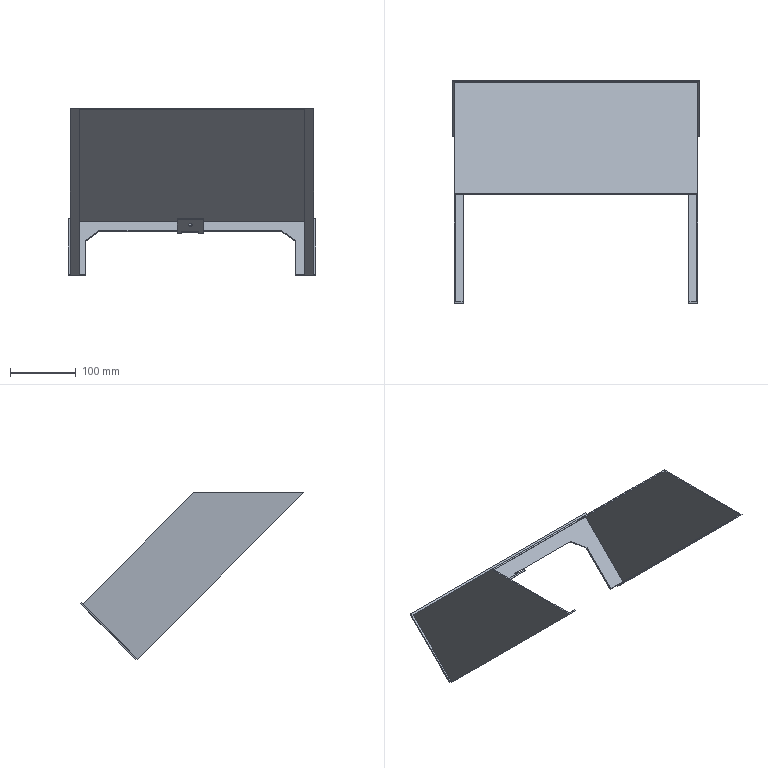Component | SolidWorks | GeneralAssembly-1_2-1 | 2 solids | 40 faces | box 378 x 340.83 x 253.5 mm | volume 369085 mm3 | plane 38 | cylinder 2 | commonest cylinder face diameters 6 x2
build123d program:
from build123d import *

# Parameters (mm, degrees)
EXTRUDE_THIN1_DEPTH = 240
BOSS_EXTRUDE1_DEPTH = 2
BOSS_EXTRUDE2_DEPTH = 2
SKETCH4_W           = 12
SKETCH4_H           = 2
BOSS_EXTRUDE3_DEPTH = 118.5
CUT_EXTRUDE1_DEPTH  = 368
BOSS_EXTRUDE4_DEPTH = 2
SKETCH7_W           = 40
SKETCH7_H           = 30
BOSS_EXTRUDE5_DEPTH = 4
SKETCH8_W           = 26
SKETCH8_H           = 5
CUT_EXTRUDE2_DEPTH  = 2
SKETCH9_W           = 28
SKETCH9_H           = 2
CUT_EXTRUDE3_DEPTH  = 40
SKETCH10_R          = 3
CUT_EXTRUDE4_DEPTH  = 2


with BuildPart() as part:
    # Sketch1 → Extrude-Thin1 (new body)
    with BuildSketch(Plane.XY):
        Polygon((-40.552, -97.131), (-54.552, -97.131), (-54.552, 21.369), (317.448, 21.369), (317.448, -97.131), (303.448, -97.131), (303.448, -95.131), (315.448, -95.131), (315.448, 19.369), (-52.552, 19.369), (-52.552, -95.131), (-40.552, -95.131), align=None)
    extrude(amount=EXTRUDE_THIN1_DEPTH)

    # Sketch2 → Boss-Extrude1 (add)
    with BuildSketch(Plane(origin=(317.448, 0, 0), x_dir=(0, 0, -1), z_dir=(1, 0, 0))):
        Polygon((-240, 21.369), (-358.5, -97.131), (-240, -97.131), align=None)
    extrude(amount=-BOSS_EXTRUDE1_DEPTH)

    # Sketch3 → Boss-Extrude2 (add)
    with BuildSketch(Plane.ZY.offset(54.552)):
        Polygon((240, 21.369), (358.5, -97.131), (240, -97.131), align=None)
    extrude(amount=-BOSS_EXTRUDE2_DEPTH)

    # Sketch4 → Boss-Extrude3 (add)
    with BuildSketch(Plane.XY.offset(240)):
        with Locations((-46.552, -96.131)):
            Rectangle(SKETCH4_W, SKETCH4_H)
        with Locations((309.448, -96.131)):
            Rectangle(SKETCH4_W, SKETCH4_H)
    extrude(amount=BOSS_EXTRUDE3_DEPTH)

    # Sketch5 → Cut-Extrude1 (cut)
    with BuildSketch(Plane(origin=(315.448, 0, 0), x_dir=(0, 0, -1), z_dir=(1, 0, 0))):
        Polygon((-358.5, -97.131), (-356.5, -95.131), (-358.5, -95.131), align=None)
    extrude(amount=-CUT_EXTRUDE1_DEPTH, mode=Mode.SUBTRACT)


with BuildPart() as body_2:
    # Sketch6 → Boss-Extrude4 (new body)
    with BuildSketch(Plane(origin=(0, 0, 0), x_dir=(-1, 0, 0), z_dir=(0, 0, -1))):
        Polygon((31.552, -95.131), (57.552, -95.131), (57.552, 24.369), (-320.448, 24.369), (-320.448, -95.131), (-289.448, -95.131), (-289.448, -22.631), (-268.448, -1.631), (10.552, -1.631), (31.552, -22.631), align=None)
    extrude(amount=BOSS_EXTRUDE4_DEPTH)

    # Sketch7 → Boss-Extrude5 (add)
    with BuildSketch(Plane.XZ.offset(1.631)):
        with Locations((128.948, 13)):
            Rectangle(SKETCH7_W, SKETCH7_H)
    extrude(amount=BOSS_EXTRUDE5_DEPTH)

    # Sketch8 → Cut-Extrude2 (cut)
    with BuildSketch(Plane(origin=(0, -5.631, 0), x_dir=(-1, 0, 0), z_dir=(0, -1, 0))):
        with Locations((-128.948, -0.5)):
            Rectangle(SKETCH8_W, SKETCH8_H)
    extrude(amount=-CUT_EXTRUDE2_DEPTH, mode=Mode.SUBTRACT)

    # Sketch9 → Cut-Extrude3 (cut)
    with BuildSketch(Plane.ZY.offset(-108.948)):
        with Locations((14, -2.631)):
            Rectangle(SKETCH9_W, SKETCH9_H)
    extrude(amount=-CUT_EXTRUDE3_DEPTH, mode=Mode.SUBTRACT)

    # Sketch10 → Cut-Extrude4 (cut)
    with BuildSketch(Plane(origin=(0, -5.631, 0), x_dir=(-1, 0, 0), z_dir=(0, -1, 0))):
        with Locations(Location((-128.948, -16.57, 0), (0, 0, 180))):
            Circle(SKETCH10_R)
    extrude(amount=-CUT_EXTRUDE4_DEPTH, mode=Mode.SUBTRACT)


solid = Compound([part.part, body_2.part])

# Placed as in the assembly
solid = solid.moved(Location((30.377, 404.357, -532.776), (45, 0, 0)))